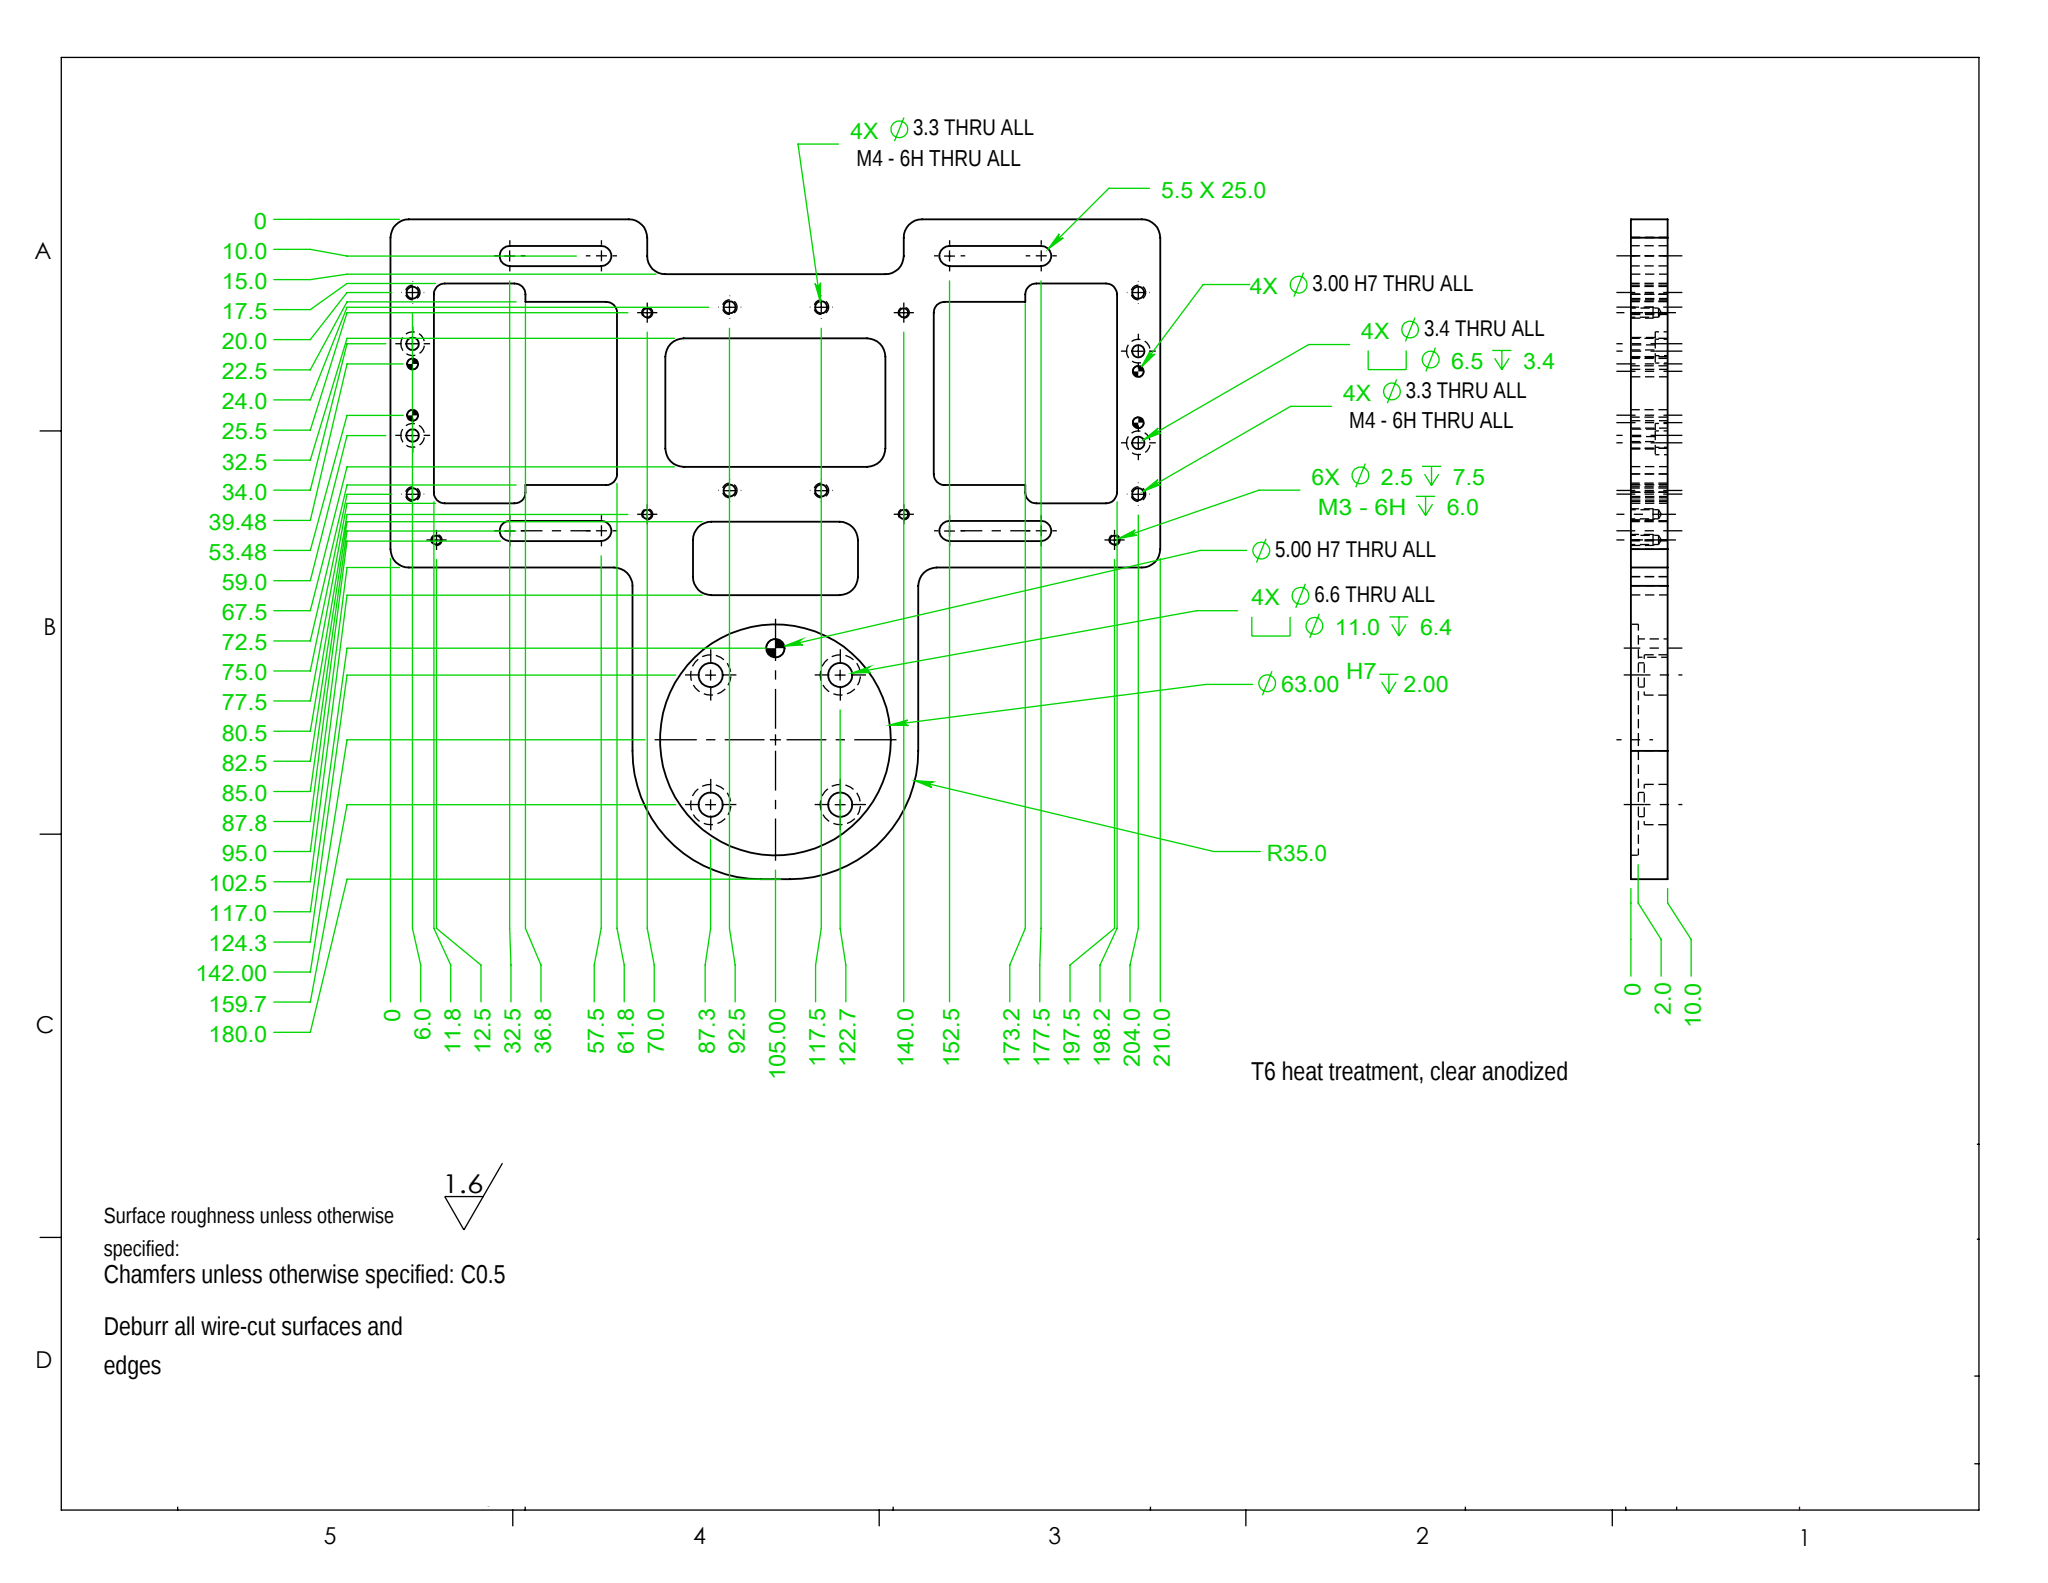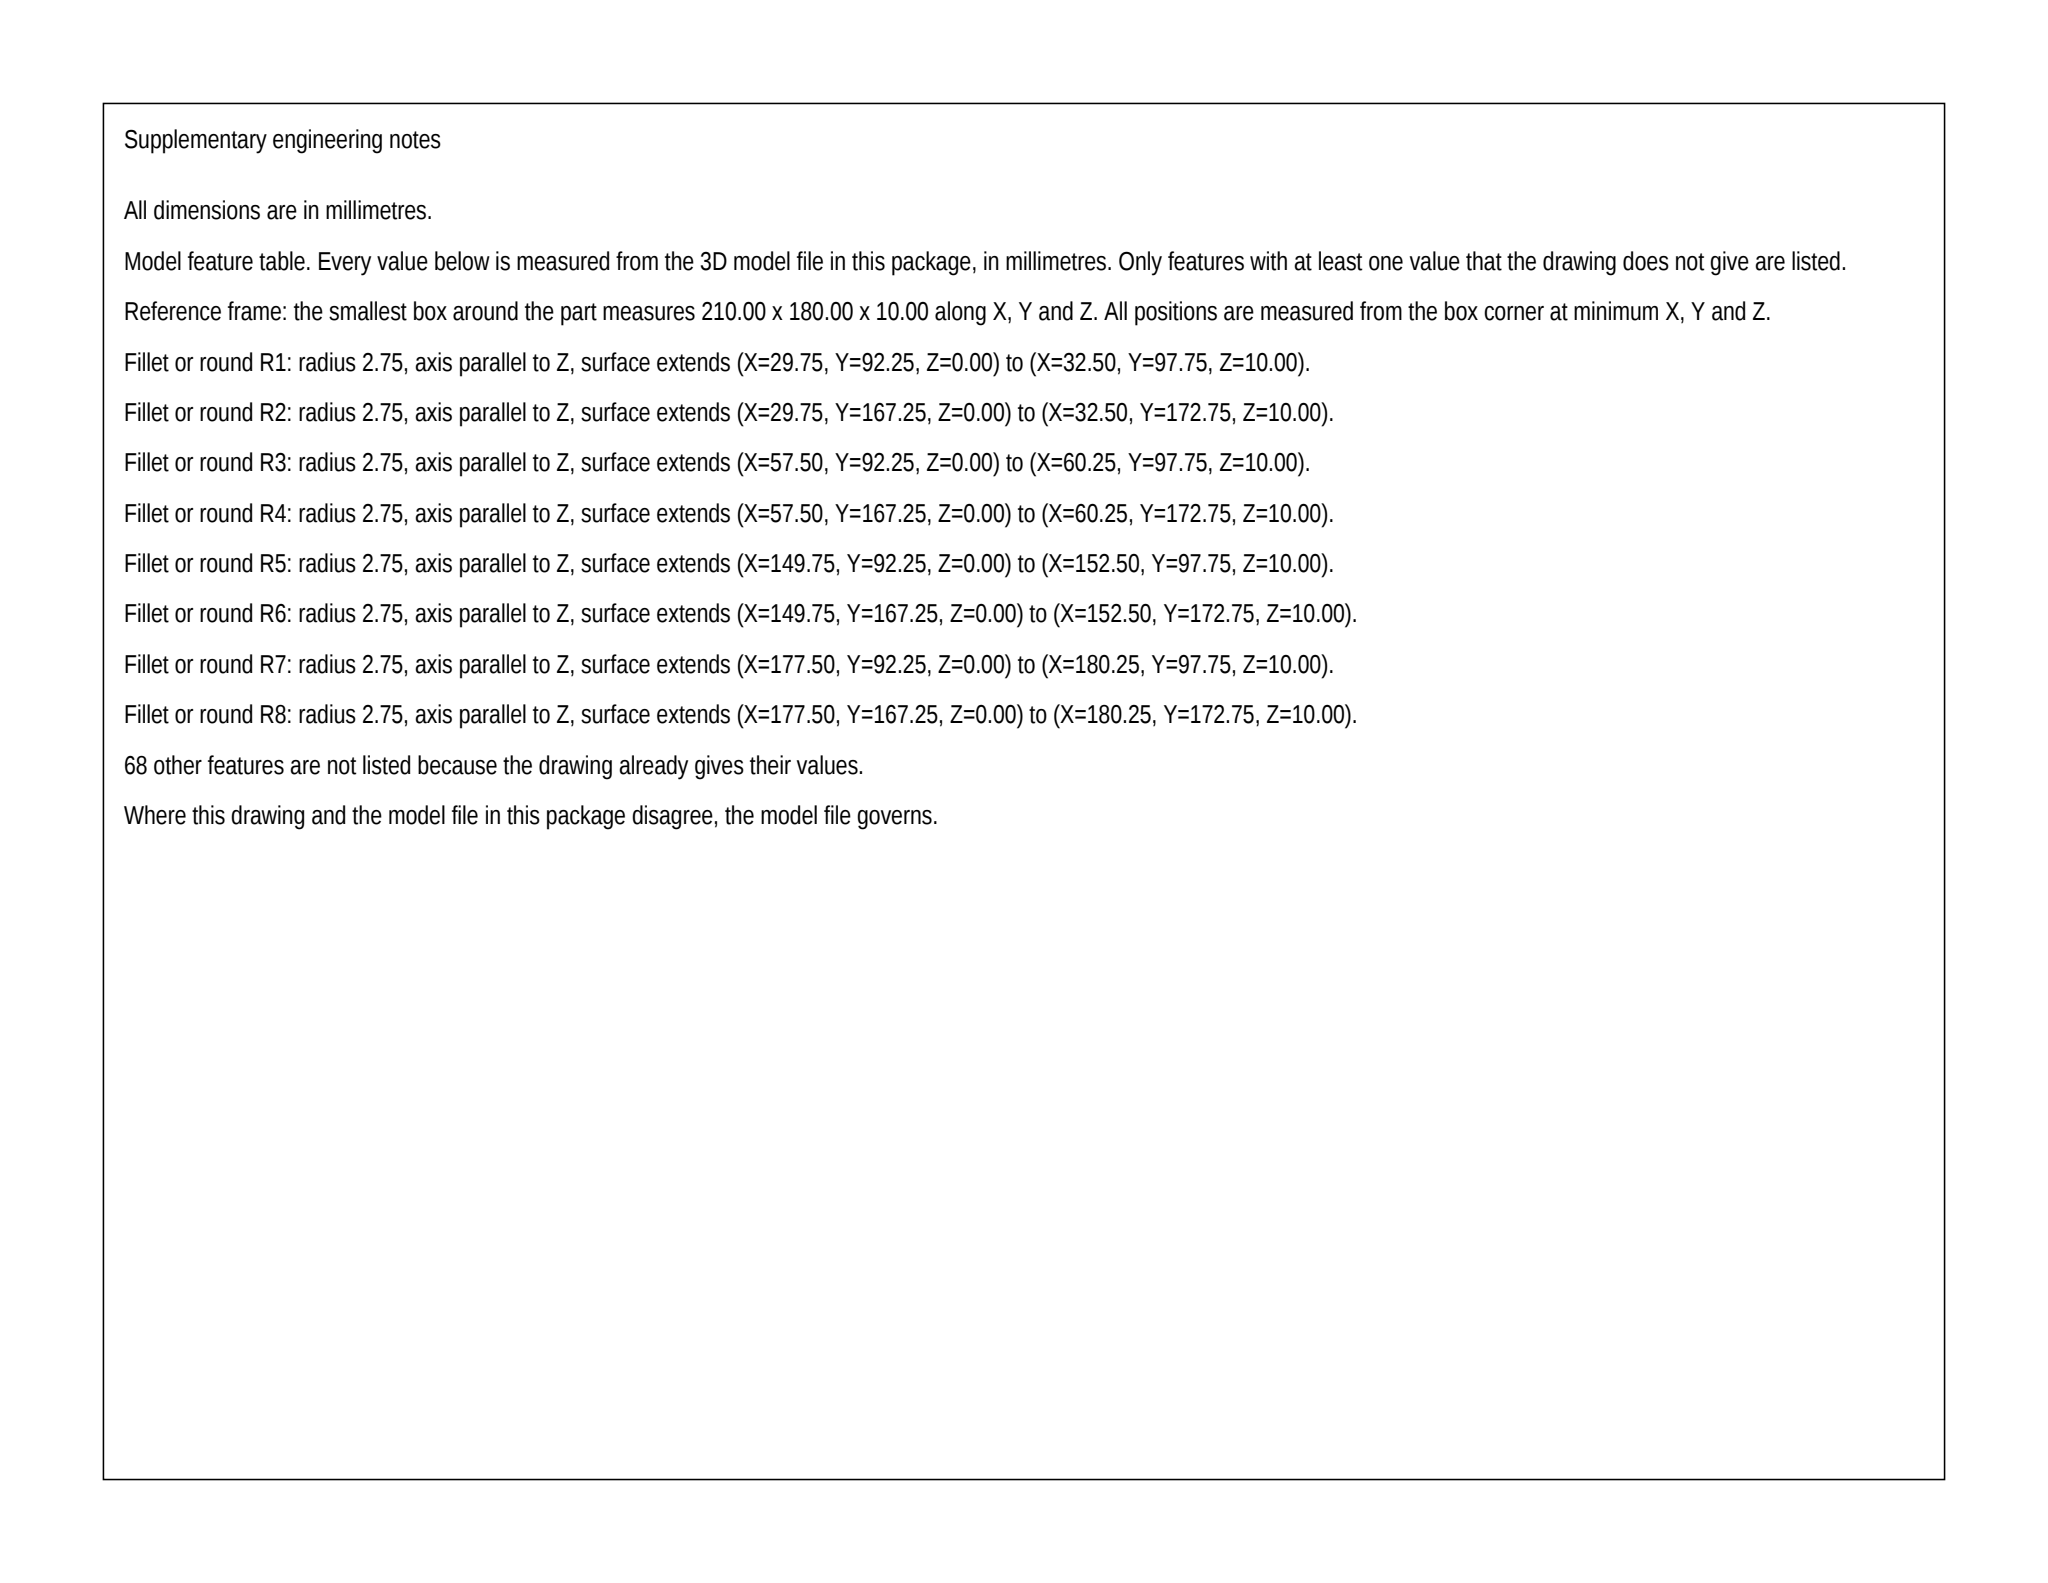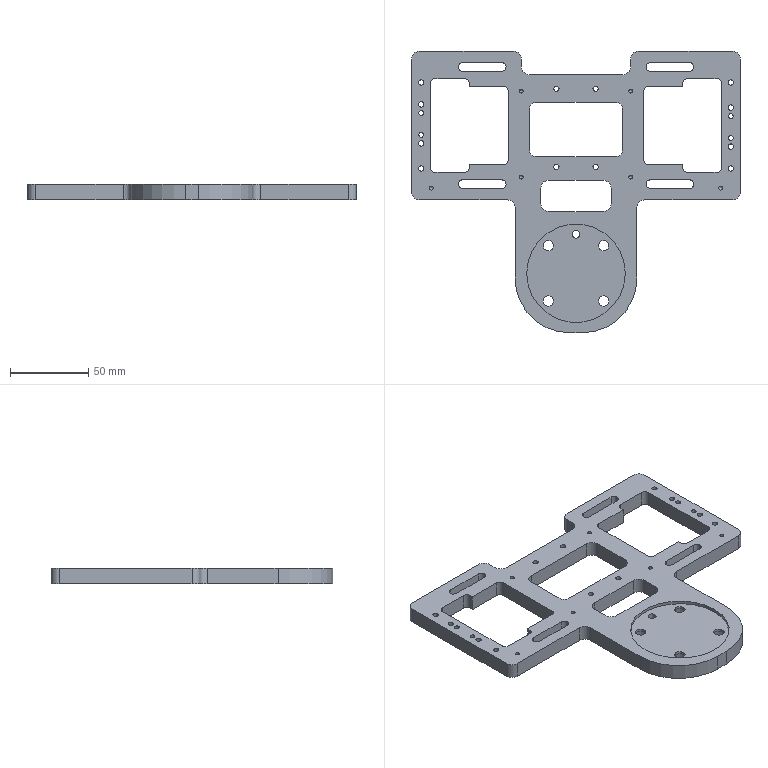Part | SolidWorks | mm | 1 solid | 183 faces | box 210 x 180 x 10 mm | volume 148216 mm3 | cylinder 116 | plane 55 | cone 12 | commonest cylinder face diameters 10 x18 3.3 x16 2.5 x12 5.5 x12 6 x12 3 x8 6.5 x8 3.4 x8
Drawing notes:
CTR RECT THRU POCKET 60 WIDE: X75 TO X135 (ORD FROM LH EDGE) | from the solid: axis_planes x=75 & x=135 with pocket cnr cyls d10 at (80,117.5),(130,142.5); y planes 112.5/147.5 = 32.5/67.5 from top
LWR ROUNDED THRU POCKET 45 WIDE: X82.5 TO X127.5 | from the solid: axis_planes x=82.5 & x=127.5; cnr cyls d10 at (87.5,82.5),(122.5,92.5); y planes 77.5/97.5 = 102.5/82.5 from top
RH OUTLINE STEP INNER CNR AT X148.2 | from the solid: axis_plane x=148.2 (mirror of dimensioned x=61.8); R3 cnr cyls d6 at (151.2,110.5),(151.2,154.5)
R35 BOSS FLANKS X66 & X144; R35 CTRS X101 & X109, 145 FR TOP | from the solid: axis_planes x=66 & x=144; cyl d70 (=R35) axes at (101,35) and (109,35); 180-35=145 from top datum
RH 2X Ø3.00 H7 AT X204: 41.5 & 55.5 FROM TOP | from the solid: cyl d3.0 at (204,138.5) & (204,124.5); 180-138.5=41.5, 180-124.5=55.5
RH 2X Ø3.4 CBORE Ø6.5 DP 3.4 AT X204: 36.0 & 61.0 FROM TOP | from the solid: cyl d3.4 at (204,144) & (204,119) with d6.5 c'bores same axes; 180-144=36, 180-119=61
CTR 2X Ø3.3 M4-6H AT X92.5 & X117.5, LWR ROW 74.0 FROM TOP | from the solid: cyl d3.3 at (92.5,106) & (117.5,106); 180-106=74.0
2X Ø2.5 DP 7.5 / M3-6H AT X12.5 & X197.5: 87.5 FROM TOP | from the solid: cyl d2.5 len7.5 at (12.5,92.5) & (197.5,92.5); 180-92.5=87.5
UNSPEC CNR RADII: R5 OUTER PROFILE & THRU POCKETS, R3 OTHERS | from the solid: cnr cyls d10 (R5) at outer profile (5,90),(205,175),(61,80),(75,170) & pockets (80,117.5),(87.5,82.5); cyls d6 (R3) at recesses (14.8,105.5),(176.2,159.5) & steps (58.8,110.5),(151.2,154.5)
Ø63 H7 DP 2.0 FROM 0 FACE; ALL C'BORES FROM 10.0 FACE, EDGE VIEW | from the solid: z planes: recess floor z=8.0 (10-2) under d63; c'bore floors z=6.4 (4X d11) and z=3.4 (4X d6.5) measured from z=0 face
build123d program:
from build123d import *

# Parameters (mm, degrees)
BOSS_EXTRUDE1_DEPTH                             = 10
SKETCH2_R                                       = 31.5
CUT_EXTRUDE1_DEPTH                              = 2
M6_HEX_SOCKET_HEAD_CAP_SCREW_CBORE1_D           = 6.6
M6_HEX_SOCKET_HEAD_CAP_SCREW_CBORE1_CBORE_D     = 11
M6_HEX_SOCKET_HEAD_CAP_SCREW_CBORE1_CBORE_DEPTH = 6.4
SIZE_MM_DOWEL_PIN_HOLE_0_D                      = 5
SKETCH9_W                                       = 70
SKETCH9_H                                       = 15
BOSS_EXTRUDE2_DEPTH                             = 10
SKETCH10_W                                      = 50
SKETCH10_H                                      = 50
CUT_EXTRUDE3_DEPTH                              = 170.355
FILLET3_R                                       = 3
CUT_EXTRUDE4_DEPTH                              = 170.355
FILLET4_R                                       = 5
SKETCH12_W                                      = 60
SKETCH12_H                                      = 35
SKETCH12_W_2                                    = 45
SKETCH12_H_2                                    = 20
CUT_EXTRUDE5_DEPTH                              = 170.355
FILLET5_R                                       = 5
FILLET6_R                                       = 35
SKETCH13_W                                      = 25
SKETCH13_H                                      = 60
CUT_EXTRUDE6_DEPTH                              = 170.355
FILLET7_R                                       = 3
M3_HEX_SOCKET_HEAD_CAP_SCREW_CBORE1_D           = 3.4
M3_HEX_SOCKET_HEAD_CAP_SCREW_CBORE1_CBORE_D     = 6.5
M3_HEX_SOCKET_HEAD_CAP_SCREW_CBORE1_CBORE_DEPTH = 3.4
SIZE_MM_DOWEL_PIN_HOLE_1_D                      = 3
M3_TAPPED_HOLE1_D                               = 2.5
M3_TAPPED_HOLE1_DEPTH                           = 7.5
M3_TAPPED_HOLE1_TIP                             = 0.7511
M4_TAPPED_HOLE1_D                               = 3.3
M4_TAPPED_HOLE2_D                               = 3.3


with BuildPart() as part:
    # Sketch1 → Boss-Extrude1 (new body)
    with BuildSketch(Plane.XY):
        Polygon((-105, 32.5), (105, 32.5), (105, -32.5), (39, -32.5), (39, -132.5), (-39, -132.5), (-39, -32.5), (-105, -32.5), align=None)
    extrude(amount=BOSS_EXTRUDE1_DEPTH)

    # Sketch2 → Cut-Extrude1 (cut)
    with BuildSketch(Plane.XY.offset(10)):
        with Locations((0, -94.5)):
            Circle(SKETCH2_R)
    extrude(amount=-CUT_EXTRUDE1_DEPTH, mode=Mode.SUBTRACT)

    # M6 Hex Socket Head Cap Screw CBORE1 (through all)
    with Locations(Plane(origin=(0, 0, 0), x_dir=(-1, 0, 0), z_dir=(0, 0, -1))):
        with Locations((17.678, -76.822), (17.678, -112.178), (-17.678, -112.178), (-17.678, -76.822)):
            CounterBoreHole(M6_HEX_SOCKET_HEAD_CAP_SCREW_CBORE1_D / 2, M6_HEX_SOCKET_HEAD_CAP_SCREW_CBORE1_CBORE_D / 2, M6_HEX_SOCKET_HEAD_CAP_SCREW_CBORE1_CBORE_DEPTH)

    # Size mm Dowel Pin Hole 0 (through all)
    with Locations(Plane(origin=(0, 0, 0), x_dir=(-1, 0, 0), z_dir=(0, 0, -1))):
        with Locations((0, -69.5)):
            Hole(SIZE_MM_DOWEL_PIN_HOLE_0_D / 2)

    # Sketch9 → Boss-Extrude2 (add)
    with BuildSketch(Plane.XY.offset(10)):
        with Locations((-70, 40)):
            Rectangle(SKETCH9_W, SKETCH9_H)
        with Locations((-70, -40)):
            Rectangle(SKETCH9_W, SKETCH9_H)
        with Locations((70, 40)):
            Rectangle(SKETCH9_W, SKETCH9_H)
        with Locations((70, -40)):
            Rectangle(SKETCH9_W, SKETCH9_H)
    extrude(amount=-BOSS_EXTRUDE2_DEPTH)

    # Sketch10 → Cut-Extrude3 (cut, through all)
    with BuildSketch(Plane.XY.offset(10)):
        with Locations((-68.2, 0)):
            Rectangle(SKETCH10_W, SKETCH10_H)
        with Locations((68.2, 0)):
            Rectangle(SKETCH10_W, SKETCH10_H)
    extrude(amount=-CUT_EXTRUDE3_DEPTH, mode=Mode.SUBTRACT)

    # Fillet3
    fillet3_edges = [part.edges().sort_by_distance(p)[0] for p in [
        (-43.2, 25, 5),
        (-43.2, -25, 5),
        (43.2, 25, 5),
        (43.2, -25, 5),
    ]]
    fillet(fillet3_edges, radius=FILLET3_R)

    # Sketch11 → Cut-Extrude4 (cut, through all)
    with BuildSketch(Plane.XY.offset(10)):
        with BuildLine():
            Line((-72.5, 40.25), (-47.5, 40.25))
            ThreePointArc((-47.5, 40.25), (-44.75, 37.5), (-47.5, 34.75))
            Line((-47.5, 34.75), (-72.5, 34.75))
            ThreePointArc((-72.5, 34.75), (-75.25, 37.5), (-72.5, 40.25))
        make_face()
        with BuildLine():
            Line((-72.5, -34.75), (-47.5, -34.75))
            ThreePointArc((-47.5, -34.75), (-44.75, -37.5), (-47.5, -40.25))
            Line((-47.5, -40.25), (-72.5, -40.25))
            ThreePointArc((-72.5, -40.25), (-75.25, -37.5), (-72.5, -34.75))
        make_face()
        with BuildLine():
            Line((47.5, 40.25), (72.5, 40.25))
            ThreePointArc((72.5, 40.25), (75.25, 37.5), (72.5, 34.75))
            Line((72.5, 34.75), (47.5, 34.75))
            ThreePointArc((47.5, 34.75), (44.75, 37.5), (47.5, 40.25))
        make_face()
        with BuildLine():
            Line((47.5, -34.75), (72.5, -34.75))
            ThreePointArc((72.5, -34.75), (75.25, -37.5), (72.5, -40.25))
            Line((72.5, -40.25), (47.5, -40.25))
            ThreePointArc((47.5, -40.25), (44.75, -37.5), (47.5, -34.75))
        make_face()
    extrude(amount=-CUT_EXTRUDE4_DEPTH, mode=Mode.SUBTRACT)

    # Fillet4
    fillet4_edges = [part.edges().sort_by_distance(p)[0] for p in [
        (105, -47.5, 5),
        (39, -47.5, 5),
        (-105, 47.5, 5),
        (-35, 47.5, 5),
        (-35, 32.5, 5),
        (105, 47.5, 5),
        (35, 32.5, 5),
        (35, 47.5, 5),
        (-105, -47.5, 5),
        (-39, -47.5, 5),
    ]]
    fillet(fillet4_edges, radius=FILLET4_R)

    # Sketch12 → Cut-Extrude5 (cut, through all)
    with BuildSketch(Plane.XY.offset(10)):
        with Locations((0, -2.5)):
            Rectangle(SKETCH12_W, SKETCH12_H)
        with Locations((0, -45)):
            Rectangle(SKETCH12_W_2, SKETCH12_H_2)
    extrude(amount=-CUT_EXTRUDE5_DEPTH, mode=Mode.SUBTRACT)

    # Fillet5
    fillet5_edges = [part.edges().sort_by_distance(p)[0] for p in [
        (-30, -20, 5),
        (-30, 15, 5),
        (30, 15, 5),
        (30, -20, 5),
        (-22.5, -55, 5),
        (-22.5, -35, 5),
        (22.5, -35, 5),
        (22.5, -55, 5),
    ]]
    fillet(fillet5_edges, radius=FILLET5_R)

    # Fillet6
    fillet6_edges = [part.edges().sort_by_distance(p)[0] for p in [
        (39, -132.5, 5),
        (-39, -132.5, 5),
    ]]
    fillet(fillet6_edges, radius=FILLET6_R)

    # Sketch13 → Cut-Extrude6 (cut, through all)
    with BuildSketch(Plane.XY.offset(10)):
        with Locations((80.7, 0)):
            Rectangle(SKETCH13_W, SKETCH13_H)
        with Locations((-80.7, 0)):
            Rectangle(SKETCH13_W, SKETCH13_H)
    extrude(amount=-CUT_EXTRUDE6_DEPTH, mode=Mode.SUBTRACT)

    # Fillet7
    fillet7_edges = [part.edges().sort_by_distance(p)[0] for p in [
        (93.2, 30, 5),
        (68.2, -30, 5),
        (93.2, -30, 5),
        (68.2, 30, 5),
        (-93.2, -30, 5),
        (-68.2, 30, 5),
        (-93.2, 30, 5),
        (-68.2, -30, 5),
    ]]
    fillet(fillet7_edges, radius=FILLET7_R)

    # M3 Hex Socket Head Cap Screw CBORE1 (through all)
    with Locations(Plane(origin=(0, 0, 0), x_dir=(-1, 0, 0), z_dir=(0, 0, -1))):
        with Locations((-99, -13.5), (-99, 11.5), (99, -11.475), (99, 13.525)):
            CounterBoreHole(M3_HEX_SOCKET_HEAD_CAP_SCREW_CBORE1_D / 2, M3_HEX_SOCKET_HEAD_CAP_SCREW_CBORE1_CBORE_D / 2, M3_HEX_SOCKET_HEAD_CAP_SCREW_CBORE1_CBORE_DEPTH)

    # Size mm Dowel Pin Hole 1 (through all)
    with Locations(Plane(origin=(0, 0, 0), x_dir=(-1, 0, 0), z_dir=(0, 0, -1))):
        with Locations((99, 8.025), (99, -5.975), (-99, -8), (-99, 6)):
            Hole(SIZE_MM_DOWEL_PIN_HOLE_1_D / 2)

    # M3 Tapped Hole1
    with Locations(Plane.XY.offset(10)):
        with Locations((-35, -33), (35, -33), (-35, 22), (35, 22), (-92.5, -40), (92.5, -40)):
            Hole(M3_TAPPED_HOLE1_D / 2, depth=M3_TAPPED_HOLE1_DEPTH)
            with Locations((0, 0, -(M3_TAPPED_HOLE1_DEPTH + M3_TAPPED_HOLE1_TIP / 2))):  # 118° drill point
                Cone(0, M3_TAPPED_HOLE1_D / 2, M3_TAPPED_HOLE1_TIP, mode=Mode.SUBTRACT)

    # M4 Tapped Hole1 (through all)
    with Locations(Plane.XY.offset(10)):
        with Locations((-12.5, 23.5), (12.5, 23.5), (-12.5, -26.5), (12.5, -26.5)):
            Hole(M4_TAPPED_HOLE1_D / 2)

    # M4 Tapped Hole2 (through all)
    with Locations(Plane.XY.offset(10)):
        with Locations((99, 27.5), (99, -27.5), (-99, -27.5), (-99, 27.5)):
            Hole(M4_TAPPED_HOLE2_D / 2)


solid = part.part